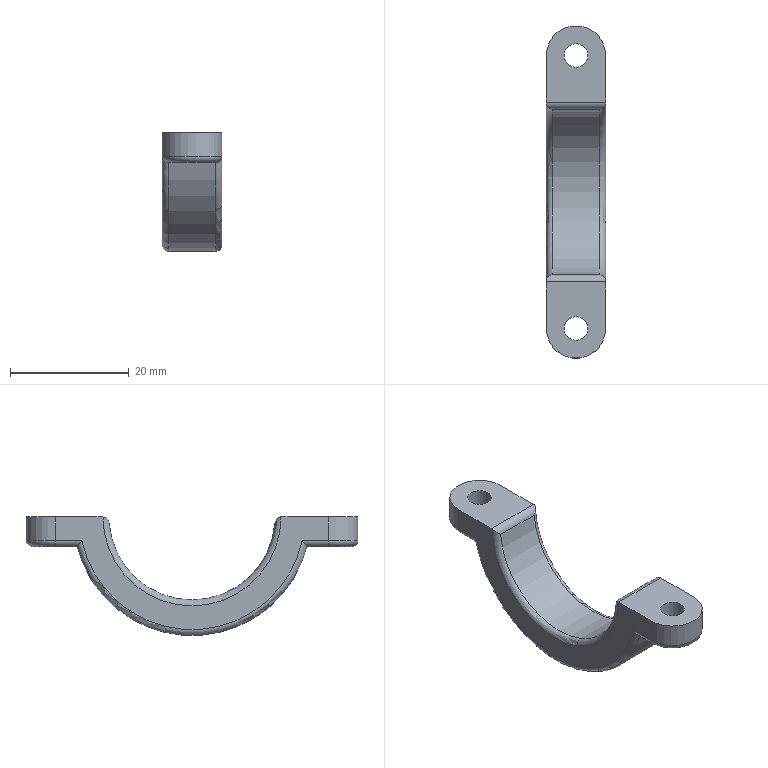Component | NX | CON_CAP | 1 solid | 24 faces | volume 3736 mm3 | cylinder 12 | plane 6 | torus 6 | commonest cylinder face diameters 2 x4 10 x2 4 x2 2.4 x2 40 x1 28 x1